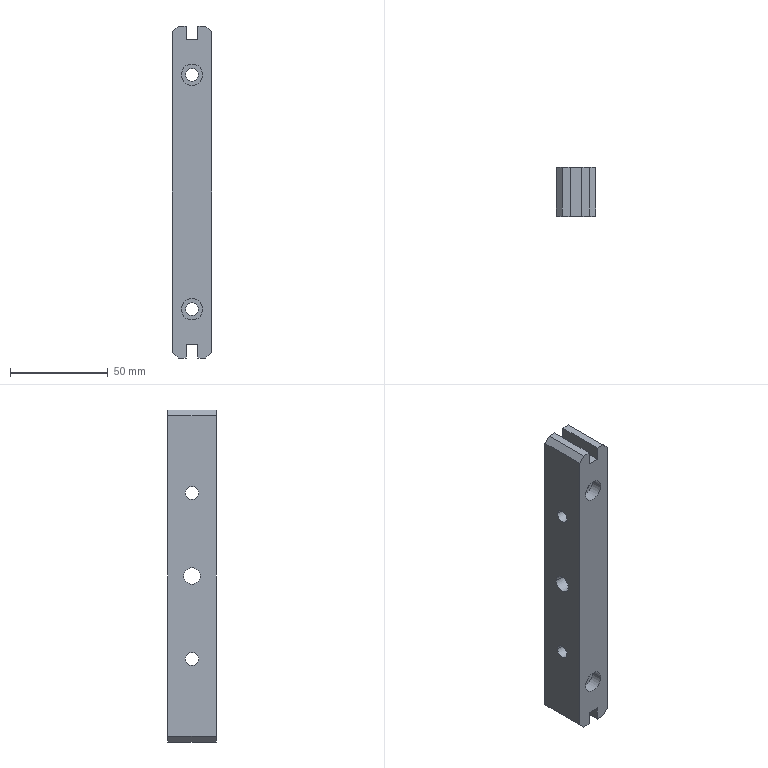Component | SolidWorks | F1-1 | 1 solid | 34 faces | box 20 x 25 x 170 mm | volume 77422 mm3 | plane 20 | cylinder 14 | commonest cylinder face diameters 11 x4 6.6 x4 6.8 x4 8.5 x2
build123d program:
from build123d import *

# Parameters (mm, degrees)
SKETCH1_W                                       = 20
SKETCH1_H                                       = 170
BOSS_EXTRUDE1_DEPTH                             = 25
SKETCH2_W                                       = 6
SKETCH2_H                                       = 7
CUT_EXTRUDE1_DEPTH                              = 1554.867
SKETCH3_R                                       = 4.25
CUT_EXTRUDE2_DEPTH                              = 227.014
M8_TAPPED_HOLE1_D                               = 6.8
M6_HEX_SOCKET_HEAD_CAP_SCREW_CBORE1_D           = 6.6
M6_HEX_SOCKET_HEAD_CAP_SCREW_CBORE1_CBORE_D     = 11
M6_HEX_SOCKET_HEAD_CAP_SCREW_CBORE1_CBORE_DEPTH = 6
CHAMFER1_SIZE                                   = 3


with BuildPart() as part:
    # Sketch1 → Boss-Extrude1 (new body)
    with BuildSketch(Plane.XY):
        with Locations((-1527.472, 138.735)):
            Rectangle(SKETCH1_W, SKETCH1_H)
    extrude(amount=BOSS_EXTRUDE1_DEPTH)

    # Sketch2 → Cut-Extrude1 (cut, through all)
    with BuildSketch(Plane.XY.offset(25)):
        with Locations((-1527.472, 220.235)):
            Rectangle(SKETCH2_W, SKETCH2_H)
        with Locations((-1527.472, 57.235)):
            Rectangle(SKETCH2_W, SKETCH2_H)
    extrude(amount=-CUT_EXTRUDE1_DEPTH, mode=Mode.SUBTRACT)

    # Sketch3 → Cut-Extrude2 (cut, through all)
    with BuildSketch(Plane(origin=(-1517.472, 0, 0), x_dir=(0, 0, -1), z_dir=(1, 0, 0))):
        with Locations((-12.5, 138.735)):
            Circle(SKETCH3_R)
    extrude(amount=-CUT_EXTRUDE2_DEPTH, mode=Mode.SUBTRACT)

    # M8 Tapped Hole1 (through all)
    with Locations(Plane(origin=(-1517.472, 0, 0), x_dir=(0, 0, -1), z_dir=(1, 0, 0))):
        with Locations((-12.5, 181.235), (-12.5, 96.235)):
            Hole(M8_TAPPED_HOLE1_D / 2)

    # M6 Hex Socket Head Cap Screw CBORE1 (through all)
    with Locations(Plane.XY.offset(25)):
        with Locations((-1527.472, 78.735), (-1527.472, 198.735)):
            CounterBoreHole(M6_HEX_SOCKET_HEAD_CAP_SCREW_CBORE1_D / 2, M6_HEX_SOCKET_HEAD_CAP_SCREW_CBORE1_CBORE_D / 2, M6_HEX_SOCKET_HEAD_CAP_SCREW_CBORE1_CBORE_DEPTH)

    # Chamfer1
    chamfer1_edges = [part.edges().sort_by_distance(p)[0] for p in [
        (-1537.472, 223.735, 12.5),
        (-1517.472, 223.735, 12.5),
        (-1517.472, 53.735, 12.5),
        (-1537.472, 53.735, 12.5),
    ]]
    chamfer(chamfer1_edges, length=CHAMFER1_SIZE)


solid = part.part

# Placed as in the assembly
solid = solid.moved(Location((1803.472, 617.279, -194.735), (90, 0, 0)))